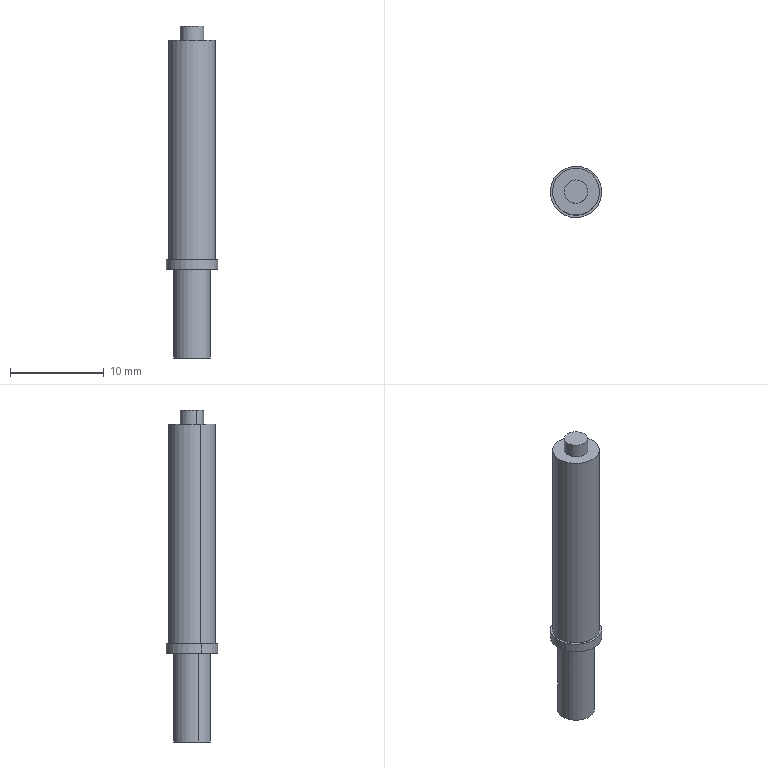Component | SolidWorks | 170423A4-ThimbleSpringGP-2T-1 | 1 solid | 17 faces | box 5.5 x 5.5 x 35.5 mm | volume 566 mm3 | cylinder 10 | plane 5 | cone 2 | commonest cylinder face diameters 2.5 x4 5 x2 5.5 x2 3.95 x2
build123d program:
from build123d import *

# Parameters (mm, degrees)
M3_TAPPED_HOLE1_D     = 2.5
M3_TAPPED_HOLE1_DEPTH = 8.5
M3_TAPPED_HOLE1_TIP   = 0.7511


with BuildPart() as part:
    # Sketch1 → Revolve1 (revolve)
    with BuildSketch(Plane(origin=(0, 0, 0), x_dir=(0, 0, -1), z_dir=(1, 0, 0))):
        Polygon((0, 35.5), (1.975, 35.5), (1.975, 26), (2.75, 26), (2.75, 25), (2.5, 25), (2.5, 1.5), (1.25, 1.5), (1.25, 0), (0, 0), align=None)
    revolve(axis=Axis((0, 0, 0), (0, 1, 0)))

    # M3 Tapped Hole1
    with Locations(Plane(origin=(0, 35.5, 0), x_dir=(-1, 0, 0), z_dir=(0, 1, 0))):
        with Locations((0, 0)):
            Hole(M3_TAPPED_HOLE1_D / 2, depth=M3_TAPPED_HOLE1_DEPTH)
            with Locations((0, 0, -(M3_TAPPED_HOLE1_DEPTH + M3_TAPPED_HOLE1_TIP / 2))):  # 118° drill point
                Cone(0, M3_TAPPED_HOLE1_D / 2, M3_TAPPED_HOLE1_TIP, mode=Mode.SUBTRACT)


solid = part.part

# Placed as in the assembly
solid = solid.moved(Location((66.187, 31.389, -54.574), (-90, 0, 0)))
STEP:
#1=COLOUR_RGB('',0.7922,0.8196,0.9333);
#2=FILL_AREA_STYLE_COLOUR('',#1);
#3=FILL_AREA_STYLE('',(#2));
#4=SURFACE_STYLE_FILL_AREA(#3);
#5=SURFACE_SIDE_STYLE('',(#4));
#6=SURFACE_STYLE_USAGE(.BOTH.,#5);
#7=PRESENTATION_STYLE_ASSIGNMENT((#6));
#8=CARTESIAN_POINT('',(2.651,1.254,-3.212));
#9=VERTEX_POINT('',#8);
#10=CARTESIAN_POINT('',(2.56,1.217,-3.212));
#11=VERTEX_POINT('',#10);
#12=CARTESIAN_POINT('',(2.606,1.236,-3.212));
#13=DIRECTION('',(-0.,0.,-1.));
#14=DIRECTION('',(-0.9265,-0.3763,0.));
#15=AXIS2_PLACEMENT_3D('',#12,#13,#14);
#16=CIRCLE('',#15,0.04921);
#17=EDGE_CURVE('',#9,#11,#16,.T.);
#18=ORIENTED_EDGE('',*,*,#17,.F.);
#19=CARTESIAN_POINT('',(2.651,1.254,-3.546));
#20=VERTEX_POINT('',#19);
#21=CARTESIAN_POINT('',(2.651,1.254,-3.546));
#22=DIRECTION('',(-0.,0.,-1.));
#23=VECTOR('',#22,39.37);
#24=LINE('',#21,#23);
#25=EDGE_CURVE('',#9,#20,#24,.T.);
#26=ORIENTED_EDGE('',*,*,#25,.T.);
#27=CARTESIAN_POINT('',(2.56,1.217,-3.546));
#28=VERTEX_POINT('',#27);
#29=CARTESIAN_POINT('',(2.606,1.236,-3.546));
#30=DIRECTION('',(-0.,0.,-1.));
#31=DIRECTION('',(-0.9265,-0.3763,0.));
#32=AXIS2_PLACEMENT_3D('',#29,#30,#31);
#33=CIRCLE('',#32,0.04921);
#34=EDGE_CURVE('',#20,#28,#33,.T.);
#35=ORIENTED_EDGE('',*,*,#34,.T.);
#36=CARTESIAN_POINT('',(2.56,1.217,-3.546));
#37=DIRECTION('',(-0.,0.,-1.));
#38=VECTOR('',#37,39.37);
#39=LINE('',#36,#38);
#40=EDGE_CURVE('',#11,#28,#39,.T.);
#41=ORIENTED_EDGE('',*,*,#40,.F.);
#42=EDGE_LOOP('',(#18,#26,#35,#41));
#43=FACE_OUTER_BOUND('',#42,.T.);
#44=CARTESIAN_POINT('',(2.606,1.236,-3.546));
#45=DIRECTION('',(-0.,0.,-1.));
#46=DIRECTION('',(-0.9265,-0.3763,0.));
#47=AXIS2_PLACEMENT_3D('',#44,#45,#46);
#48=CYLINDRICAL_SURFACE('',#47,0.04921);
#49=ADVANCED_FACE('',(#43),#48,.F.);
#50=CARTESIAN_POINT('',(2.606,1.236,-3.182));
#51=VERTEX_POINT('',#50);
#52=CARTESIAN_POINT('',(2.56,1.217,-3.212));
#53=DIRECTION('',(-0.7942,-0.3226,-0.515));
#54=VECTOR('',#53,39.37);
#55=LINE('',#52,#54);
#56=EDGE_CURVE('',#51,#11,#55,.T.);
#57=ORIENTED_EDGE('',*,*,#56,.F.);
#58=CARTESIAN_POINT('',(2.651,1.254,-3.212));
#59=DIRECTION('',(0.7942,0.3226,-0.515));
#60=VECTOR('',#59,39.37);
#61=LINE('',#58,#60);
#62=EDGE_CURVE('',#51,#9,#61,.T.);
#63=ORIENTED_EDGE('',*,*,#62,.T.);
#64=ORIENTED_EDGE('',*,*,#17,.T.);
#65=EDGE_LOOP('',(#57,#63,#64));
#66=FACE_OUTER_BOUND('',#65,.T.);
#67=CARTESIAN_POINT('',(2.606,1.236,-3.212));
#68=DIRECTION('',(-0.,0.,-1.));
#69=DIRECTION('',(-0.9265,-0.3763,0.));
#70=AXIS2_PLACEMENT_3D('',#67,#68,#69);
#71=CONICAL_SURFACE('',#70,0.04921,1.03);
#72=ADVANCED_FACE('',(#66),#71,.F.);
#73=CARTESIAN_POINT('',(2.651,1.254,-2.208));
#74=VERTEX_POINT('',#73);
#75=CARTESIAN_POINT('',(2.56,1.217,-2.208));
#76=VERTEX_POINT('',#75);
#77=CARTESIAN_POINT('',(2.606,1.236,-2.208));
#78=DIRECTION('',(0.,-0.,1.));
#79=DIRECTION('',(0.9265,0.3763,0.));
#80=AXIS2_PLACEMENT_3D('',#77,#78,#79);
#81=CIRCLE('',#80,0.04921);
#82=EDGE_CURVE('',#74,#76,#81,.T.);
#83=ORIENTED_EDGE('',*,*,#82,.T.);
#84=CARTESIAN_POINT('',(2.56,1.217,-2.149));
#85=VERTEX_POINT('',#84);
#86=CARTESIAN_POINT('',(2.56,1.217,-2.149));
#87=DIRECTION('',(0.,-0.,1.));
#88=VECTOR('',#87,39.37);
#89=LINE('',#86,#88);
#90=EDGE_CURVE('',#76,#85,#89,.T.);
#91=ORIENTED_EDGE('',*,*,#90,.T.);
#92=CARTESIAN_POINT('',(2.651,1.254,-2.149));
#93=VERTEX_POINT('',#92);
#94=CARTESIAN_POINT('',(2.606,1.236,-2.149));
#95=DIRECTION('',(0.,-0.,1.));
#96=DIRECTION('',(0.9265,0.3763,0.));
#97=AXIS2_PLACEMENT_3D('',#94,#95,#96);
#98=CIRCLE('',#97,0.04921);
#99=EDGE_CURVE('',#93,#85,#98,.T.);
#100=ORIENTED_EDGE('',*,*,#99,.F.);
#101=CARTESIAN_POINT('',(2.651,1.254,-2.149));
#102=DIRECTION('',(0.,-0.,1.));
#103=VECTOR('',#102,39.37);
#104=LINE('',#101,#103);
#105=EDGE_CURVE('',#74,#93,#104,.T.);
#106=ORIENTED_EDGE('',*,*,#105,.F.);
#107=EDGE_LOOP('',(#83,#91,#100,#106));
#108=FACE_OUTER_BOUND('',#107,.T.);
#109=CARTESIAN_POINT('',(2.606,1.236,-2.149));
#110=DIRECTION('',(0.,-0.,1.));
#111=DIRECTION('',(0.9265,0.3763,0.));
#112=AXIS2_PLACEMENT_3D('',#109,#110,#111);
#113=CYLINDRICAL_SURFACE('',#112,0.04921);
#114=ADVANCED_FACE('',(#108),#113,.T.);
#115=CARTESIAN_POINT('',(2.697,1.273,-3.133));
#116=VERTEX_POINT('',#115);
#117=CARTESIAN_POINT('',(2.515,1.199,-3.133));
#118=VERTEX_POINT('',#117);
#119=CARTESIAN_POINT('',(2.606,1.236,-3.133));
#120=DIRECTION('',(0.,-0.,1.));
#121=DIRECTION('',(0.9265,0.3763,0.));
#122=AXIS2_PLACEMENT_3D('',#119,#120,#121);
#123=CIRCLE('',#122,0.09843);
#124=EDGE_CURVE('',#116,#118,#123,.T.);
#125=ORIENTED_EDGE('',*,*,#124,.T.);
#126=CARTESIAN_POINT('',(2.515,1.199,-2.208));
#127=VERTEX_POINT('',#126);
#128=CARTESIAN_POINT('',(2.515,1.199,-2.149));
#129=DIRECTION('',(0.,-0.,1.));
#130=VECTOR('',#129,39.37);
#131=LINE('',#128,#130);
#132=EDGE_CURVE('',#118,#127,#131,.T.);
#133=ORIENTED_EDGE('',*,*,#132,.T.);
#134=CARTESIAN_POINT('',(2.697,1.273,-2.208));
#135=VERTEX_POINT('',#134);
#136=CARTESIAN_POINT('',(2.606,1.236,-2.208));
#137=DIRECTION('',(0.,-0.,1.));
#138=DIRECTION('',(0.9265,0.3763,0.));
#139=AXIS2_PLACEMENT_3D('',#136,#137,#138);
#140=CIRCLE('',#139,0.09843);
#141=EDGE_CURVE('',#135,#127,#140,.T.);
#142=ORIENTED_EDGE('',*,*,#141,.F.);
#143=CARTESIAN_POINT('',(2.697,1.273,-2.149));
#144=DIRECTION('',(0.,-0.,1.));
#145=VECTOR('',#144,39.37);
#146=LINE('',#143,#145);
#147=EDGE_CURVE('',#116,#135,#146,.T.);
#148=ORIENTED_EDGE('',*,*,#147,.F.);
#149=EDGE_LOOP('',(#125,#133,#142,#148));
#150=FACE_OUTER_BOUND('',#149,.T.);
#151=CARTESIAN_POINT('',(2.606,1.236,-2.149));
#152=DIRECTION('',(0.,-0.,1.));
#153=DIRECTION('',(0.9265,0.3763,0.));
#154=AXIS2_PLACEMENT_3D('',#151,#152,#153);
#155=CYLINDRICAL_SURFACE('',#154,0.09843);
#156=ADVANCED_FACE('',(#150),#155,.T.);
#157=CARTESIAN_POINT('',(2.706,1.277,-3.172));
#158=VERTEX_POINT('',#157);
#159=CARTESIAN_POINT('',(2.505,1.195,-3.172));
#160=VERTEX_POINT('',#159);
#161=CARTESIAN_POINT('',(2.606,1.236,-3.172));
#162=DIRECTION('',(0.,-0.,1.));
#163=DIRECTION('',(0.9265,0.3763,0.));
#164=AXIS2_PLACEMENT_3D('',#161,#162,#163);
#165=CIRCLE('',#164,0.1083);
#166=EDGE_CURVE('',#158,#160,#165,.T.);
#167=ORIENTED_EDGE('',*,*,#166,.T.);
#168=CARTESIAN_POINT('',(2.505,1.195,-3.133));
#169=VERTEX_POINT('',#168);
#170=CARTESIAN_POINT('',(2.505,1.195,-2.149));
#171=DIRECTION('',(0.,-0.,1.));
#172=VECTOR('',#171,39.37);
#173=LINE('',#170,#172);
#174=EDGE_CURVE('',#160,#169,#173,.T.);
#175=ORIENTED_EDGE('',*,*,#174,.T.);
#176=CARTESIAN_POINT('',(2.706,1.277,-3.133));
#177=VERTEX_POINT('',#176);
#178=CARTESIAN_POINT('',(2.606,1.236,-3.133));
#179=DIRECTION('',(0.,-0.,1.));
#180=DIRECTION('',(0.9265,0.3763,0.));
#181=AXIS2_PLACEMENT_3D('',#178,#179,#180);
#182=CIRCLE('',#181,0.1083);
#183=EDGE_CURVE('',#177,#169,#182,.T.);
#184=ORIENTED_EDGE('',*,*,#183,.F.);
#185=CARTESIAN_POINT('',(2.706,1.277,-2.149));
#186=DIRECTION('',(0.,-0.,1.));
#187=VECTOR('',#186,39.37);
#188=LINE('',#185,#187);
#189=EDGE_CURVE('',#158,#177,#188,.T.);
#190=ORIENTED_EDGE('',*,*,#189,.F.);
#191=EDGE_LOOP('',(#167,#175,#184,#190));
#192=FACE_OUTER_BOUND('',#191,.T.);
#193=CARTESIAN_POINT('',(2.606,1.236,-2.149));
#194=DIRECTION('',(0.,-0.,1.));
#195=DIRECTION('',(0.9265,0.3763,0.));
#196=AXIS2_PLACEMENT_3D('',#193,#194,#195);
#197=CYLINDRICAL_SURFACE('',#196,0.1083);
#198=ADVANCED_FACE('',(#192),#197,.T.);
#199=CARTESIAN_POINT('',(2.678,1.265,-3.546));
#200=VERTEX_POINT('',#199);
#201=CARTESIAN_POINT('',(2.534,1.207,-3.546));
#202=VERTEX_POINT('',#201);
#203=CARTESIAN_POINT('',(2.606,1.236,-3.546));
#204=DIRECTION('',(0.,-0.,1.));
#205=DIRECTION('',(0.9265,0.3763,0.));
#206=AXIS2_PLACEMENT_3D('',#203,#204,#205);
#207=CIRCLE('',#206,0.07776);
#208=EDGE_CURVE('',#200,#202,#207,.T.);
#209=ORIENTED_EDGE('',*,*,#208,.T.);
#210=CARTESIAN_POINT('',(2.534,1.207,-3.172));
#211=VERTEX_POINT('',#210);
#212=CARTESIAN_POINT('',(2.534,1.207,-2.149));
#213=DIRECTION('',(0.,-0.,1.));
#214=VECTOR('',#213,39.37);
#215=LINE('',#212,#214);
#216=EDGE_CURVE('',#202,#211,#215,.T.);
#217=ORIENTED_EDGE('',*,*,#216,.T.);
#218=CARTESIAN_POINT('',(2.678,1.265,-3.172));
#219=VERTEX_POINT('',#218);
#220=CARTESIAN_POINT('',(2.606,1.236,-3.172));
#221=DIRECTION('',(0.,-0.,1.));
#222=DIRECTION('',(0.9265,0.3763,0.));
#223=AXIS2_PLACEMENT_3D('',#220,#221,#222);
#224=CIRCLE('',#223,0.07776);
#225=EDGE_CURVE('',#219,#211,#224,.T.);
#226=ORIENTED_EDGE('',*,*,#225,.F.);
#227=CARTESIAN_POINT('',(2.678,1.265,-2.149));
#228=DIRECTION('',(0.,-0.,1.));
#229=VECTOR('',#228,39.37);
#230=LINE('',#227,#229);
#231=EDGE_CURVE('',#200,#219,#230,.T.);
#232=ORIENTED_EDGE('',*,*,#231,.F.);
#233=EDGE_LOOP('',(#209,#217,#226,#232));
#234=FACE_OUTER_BOUND('',#233,.T.);
#235=CARTESIAN_POINT('',(2.606,1.236,-2.149));
#236=DIRECTION('',(0.,-0.,1.));
#237=DIRECTION('',(0.9265,0.3763,0.));
#238=AXIS2_PLACEMENT_3D('',#235,#236,#237);
#239=CYLINDRICAL_SURFACE('',#238,0.07776);
#240=ADVANCED_FACE('',(#234),#239,.T.);
#241=CARTESIAN_POINT('',(2.606,1.236,-3.546));
#242=DIRECTION('',(-0.,0.,-1.));
#243=DIRECTION('',(-0.9265,-0.3763,0.));
#244=AXIS2_PLACEMENT_3D('',#241,#242,#243);
#245=CIRCLE('',#244,0.04921);
#246=EDGE_CURVE('',#28,#20,#245,.T.);
#247=ORIENTED_EDGE('',*,*,#246,.F.);
#248=ORIENTED_EDGE('',*,*,#34,.F.);
#249=EDGE_LOOP('',(#247,#248));
#250=FACE_BOUND('',#249,.T.);
#251=ORIENTED_EDGE('',*,*,#208,.F.);
#252=CARTESIAN_POINT('',(2.606,1.236,-3.546));
#253=DIRECTION('',(0.,-0.,1.));
#254=DIRECTION('',(0.9265,0.3763,0.));
#255=AXIS2_PLACEMENT_3D('',#252,#253,#254);
#256=CIRCLE('',#255,0.07776);
#257=EDGE_CURVE('',#202,#200,#256,.T.);
#258=ORIENTED_EDGE('',*,*,#257,.F.);
#259=EDGE_LOOP('',(#251,#258));
#260=FACE_OUTER_BOUND('',#259,.T.);
#261=CARTESIAN_POINT('',(2.606,1.236,-3.546));
#262=DIRECTION('',(-0.,0.,-1.));
#263=DIRECTION('',(-0.9265,-0.3763,-0.));
#264=AXIS2_PLACEMENT_3D('',#261,#262,#263);
#265=PLANE('',#264);
#266=ADVANCED_FACE('',(#250,#260),#265,.T.);
#267=ORIENTED_EDGE('',*,*,#216,.F.);
#268=ORIENTED_EDGE('',*,*,#257,.T.);
#269=ORIENTED_EDGE('',*,*,#231,.T.);
#270=CARTESIAN_POINT('',(2.606,1.236,-3.172));
#271=DIRECTION('',(0.,-0.,1.));
#272=DIRECTION('',(0.9265,0.3763,0.));
#273=AXIS2_PLACEMENT_3D('',#270,#271,#272);
#274=CIRCLE('',#273,0.07776);
#275=EDGE_CURVE('',#211,#219,#274,.T.);
#276=ORIENTED_EDGE('',*,*,#275,.F.);
#277=EDGE_LOOP('',(#267,#268,#269,#276));
#278=FACE_OUTER_BOUND('',#277,.T.);
#279=CARTESIAN_POINT('',(2.606,1.236,-2.149));
#280=DIRECTION('',(0.,-0.,1.));
#281=DIRECTION('',(0.9265,0.3763,0.));
#282=AXIS2_PLACEMENT_3D('',#279,#280,#281);
#283=CYLINDRICAL_SURFACE('',#282,0.07776);
#284=ADVANCED_FACE('',(#278),#283,.T.);
#285=ORIENTED_EDGE('',*,*,#225,.T.);
#286=ORIENTED_EDGE('',*,*,#275,.T.);
#287=EDGE_LOOP('',(#285,#286));
#288=FACE_BOUND('',#287,.T.);
#289=ORIENTED_EDGE('',*,*,#166,.F.);
#290=CARTESIAN_POINT('',(2.606,1.236,-3.172));
#291=DIRECTION('',(0.,-0.,1.));
#292=DIRECTION('',(0.9265,0.3763,0.));
#293=AXIS2_PLACEMENT_3D('',#290,#291,#292);
#294=CIRCLE('',#293,0.1083);
#295=EDGE_CURVE('',#160,#158,#294,.T.);
#296=ORIENTED_EDGE('',*,*,#295,.F.);
#297=EDGE_LOOP('',(#289,#296));
#298=FACE_OUTER_BOUND('',#297,.T.);
#299=CARTESIAN_POINT('',(2.678,1.265,-3.172));
#300=DIRECTION('',(-0.,0.,-1.));
#301=DIRECTION('',(-0.9265,-0.3763,-0.));
#302=AXIS2_PLACEMENT_3D('',#299,#300,#301);
#303=PLANE('',#302);
#304=ADVANCED_FACE('',(#288,#298),#303,.T.);
#305=ORIENTED_EDGE('',*,*,#174,.F.);
#306=ORIENTED_EDGE('',*,*,#295,.T.);
#307=ORIENTED_EDGE('',*,*,#189,.T.);
#308=CARTESIAN_POINT('',(2.606,1.236,-3.133));
#309=DIRECTION('',(0.,-0.,1.));
#310=DIRECTION('',(0.9265,0.3763,0.));
#311=AXIS2_PLACEMENT_3D('',#308,#309,#310);
#312=CIRCLE('',#311,0.1083);
#313=EDGE_CURVE('',#169,#177,#312,.T.);
#314=ORIENTED_EDGE('',*,*,#313,.F.);
#315=EDGE_LOOP('',(#305,#306,#307,#314));
#316=FACE_OUTER_BOUND('',#315,.T.);
#317=CARTESIAN_POINT('',(2.606,1.236,-2.149));
#318=DIRECTION('',(0.,-0.,1.));
#319=DIRECTION('',(0.9265,0.3763,0.));
#320=AXIS2_PLACEMENT_3D('',#317,#318,#319);
#321=CYLINDRICAL_SURFACE('',#320,0.1083);
#322=ADVANCED_FACE('',(#316),#321,.T.);
#323=ORIENTED_EDGE('',*,*,#183,.T.);
#324=ORIENTED_EDGE('',*,*,#313,.T.);
#325=EDGE_LOOP('',(#323,#324));
#326=FACE_OUTER_BOUND('',#325,.T.);
#327=ORIENTED_EDGE('',*,*,#124,.F.);
#328=CARTESIAN_POINT('',(2.606,1.236,-3.133));
#329=DIRECTION('',(0.,-0.,1.));
#330=DIRECTION('',(0.9265,0.3763,0.));
#331=AXIS2_PLACEMENT_3D('',#328,#329,#330);
#332=CIRCLE('',#331,0.09843);
#333=EDGE_CURVE('',#118,#116,#332,.T.);
#334=ORIENTED_EDGE('',*,*,#333,.F.);
#335=EDGE_LOOP('',(#327,#334));
#336=FACE_BOUND('',#335,.T.);
#337=CARTESIAN_POINT('',(2.706,1.277,-3.133));
#338=DIRECTION('',(0.,-0.,1.));
#339=DIRECTION('',(0.9265,0.3763,0.));
#340=AXIS2_PLACEMENT_3D('',#337,#338,#339);
#341=PLANE('',#340);
#342=ADVANCED_FACE('',(#326,#336),#341,.T.);
#343=ORIENTED_EDGE('',*,*,#132,.F.);
#344=ORIENTED_EDGE('',*,*,#333,.T.);
#345=ORIENTED_EDGE('',*,*,#147,.T.);
#346=CARTESIAN_POINT('',(2.606,1.236,-2.208));
#347=DIRECTION('',(0.,-0.,1.));
#348=DIRECTION('',(0.9265,0.3763,0.));
#349=AXIS2_PLACEMENT_3D('',#346,#347,#348);
#350=CIRCLE('',#349,0.09843);
#351=EDGE_CURVE('',#127,#135,#350,.T.);
#352=ORIENTED_EDGE('',*,*,#351,.F.);
#353=EDGE_LOOP('',(#343,#344,#345,#352));
#354=FACE_OUTER_BOUND('',#353,.T.);
#355=CARTESIAN_POINT('',(2.606,1.236,-2.149));
#356=DIRECTION('',(0.,-0.,1.));
#357=DIRECTION('',(0.9265,0.3763,0.));
#358=AXIS2_PLACEMENT_3D('',#355,#356,#357);
#359=CYLINDRICAL_SURFACE('',#358,0.09843);
#360=ADVANCED_FACE('',(#354),#359,.T.);
#361=ORIENTED_EDGE('',*,*,#141,.T.);
#362=ORIENTED_EDGE('',*,*,#351,.T.);
#363=EDGE_LOOP('',(#361,#362));
#364=FACE_OUTER_BOUND('',#363,.T.);
#365=ORIENTED_EDGE('',*,*,#82,.F.);
#366=CARTESIAN_POINT('',(2.606,1.236,-2.208));
#367=DIRECTION('',(0.,-0.,1.));
#368=DIRECTION('',(0.9265,0.3763,0.));
#369=AXIS2_PLACEMENT_3D('',#366,#367,#368);
#370=CIRCLE('',#369,0.04921);
#371=EDGE_CURVE('',#76,#74,#370,.T.);
#372=ORIENTED_EDGE('',*,*,#371,.F.);
#373=EDGE_LOOP('',(#365,#372));
#374=FACE_BOUND('',#373,.T.);
#375=CARTESIAN_POINT('',(2.697,1.273,-2.208));
#376=DIRECTION('',(0.,-0.,1.));
#377=DIRECTION('',(0.9265,0.3763,0.));
#378=AXIS2_PLACEMENT_3D('',#375,#376,#377);
#379=PLANE('',#378);
#380=ADVANCED_FACE('',(#364,#374),#379,.T.);
#381=ORIENTED_EDGE('',*,*,#90,.F.);
#382=ORIENTED_EDGE('',*,*,#371,.T.);
#383=ORIENTED_EDGE('',*,*,#105,.T.);
#384=CARTESIAN_POINT('',(2.606,1.236,-2.149));
#385=DIRECTION('',(0.,-0.,1.));
#386=DIRECTION('',(0.9265,0.3763,0.));
#387=AXIS2_PLACEMENT_3D('',#384,#385,#386);
#388=CIRCLE('',#387,0.04921);
#389=EDGE_CURVE('',#85,#93,#388,.T.);
#390=ORIENTED_EDGE('',*,*,#389,.F.);
#391=EDGE_LOOP('',(#381,#382,#383,#390));
#392=FACE_OUTER_BOUND('',#391,.T.);
#393=CARTESIAN_POINT('',(2.606,1.236,-2.149));
#394=DIRECTION('',(0.,-0.,1.));
#395=DIRECTION('',(0.9265,0.3763,0.));
#396=AXIS2_PLACEMENT_3D('',#393,#394,#395);
#397=CYLINDRICAL_SURFACE('',#396,0.04921);
#398=ADVANCED_FACE('',(#392),#397,.T.);
#399=ORIENTED_EDGE('',*,*,#99,.T.);
#400=ORIENTED_EDGE('',*,*,#389,.T.);
#401=EDGE_LOOP('',(#399,#400));
#402=FACE_OUTER_BOUND('',#401,.T.);
#403=CARTESIAN_POINT('',(2.651,1.254,-2.149));
#404=DIRECTION('',(0.,-0.,1.));
#405=DIRECTION('',(0.9265,0.3763,0.));
#406=AXIS2_PLACEMENT_3D('',#403,#404,#405);
#407=PLANE('',#406);
#408=ADVANCED_FACE('',(#402),#407,.T.);
#409=ORIENTED_EDGE('',*,*,#62,.F.);
#410=ORIENTED_EDGE('',*,*,#56,.T.);
#411=CARTESIAN_POINT('',(2.606,1.236,-3.212));
#412=DIRECTION('',(-0.,0.,-1.));
#413=DIRECTION('',(-0.9265,-0.3763,0.));
#414=AXIS2_PLACEMENT_3D('',#411,#412,#413);
#415=CIRCLE('',#414,0.04921);
#416=EDGE_CURVE('',#11,#9,#415,.T.);
#417=ORIENTED_EDGE('',*,*,#416,.T.);
#418=EDGE_LOOP('',(#409,#410,#417));
#419=FACE_OUTER_BOUND('',#418,.T.);
#420=CARTESIAN_POINT('',(2.606,1.236,-3.212));
#421=DIRECTION('',(-0.,0.,-1.));
#422=DIRECTION('',(-0.9265,-0.3763,0.));
#423=AXIS2_PLACEMENT_3D('',#420,#421,#422);
#424=CONICAL_SURFACE('',#423,0.04921,1.03);
#425=ADVANCED_FACE('',(#419),#424,.F.);
#426=ORIENTED_EDGE('',*,*,#25,.F.);
#427=ORIENTED_EDGE('',*,*,#416,.F.);
#428=ORIENTED_EDGE('',*,*,#40,.T.);
#429=ORIENTED_EDGE('',*,*,#246,.T.);
#430=EDGE_LOOP('',(#426,#427,#428,#429));
#431=FACE_OUTER_BOUND('',#430,.T.);
#432=CARTESIAN_POINT('',(2.606,1.236,-3.546));
#433=DIRECTION('',(-0.,0.,-1.));
#434=DIRECTION('',(-0.9265,-0.3763,0.));
#435=AXIS2_PLACEMENT_3D('',#432,#433,#434);
#436=CYLINDRICAL_SURFACE('',#435,0.04921);
#437=ADVANCED_FACE('',(#431),#436,.F.);
#438=CLOSED_SHELL('',(#49,#72,#114,#156,#198,#240,#266,#284,#304,#322,#342,#360,#380,#398,#408,#425,#437));
#439=MANIFOLD_SOLID_BREP('',#438);
#440=STYLED_ITEM('',(#7),#439);
#441=PRESENTATION_LAYER_ASSIGNMENT('','',(#440));
#442=CARTESIAN_POINT('',(0.,0.,0.));
#443=DIRECTION('',(0.,0.,1.));
#444=DIRECTION('',(1.,0.,0.));
#445=AXIS2_PLACEMENT_3D('',#442,#443,#444);
#446=(LENGTH_UNIT()NAMED_UNIT(*)SI_UNIT($,.METRE.));
#447=LENGTH_MEASURE_WITH_UNIT(LENGTH_MEASURE(0.0254),#446);
#448=DIMENSIONAL_EXPONENTS(1.,0.,0.,0.,0.,0.,0.);
#449=(CONVERSION_BASED_UNIT('',#447)LENGTH_UNIT()NAMED_UNIT(#448));
#450=UNCERTAINTY_MEASURE_WITH_UNIT(LENGTH_MEASURE(0.00001),#449,'','');
#451=(NAMED_UNIT(*)PLANE_ANGLE_UNIT()SI_UNIT($,.RADIAN.));
#452=(NAMED_UNIT(*)SI_UNIT($,.STERADIAN.)SOLID_ANGLE_UNIT());
#453=(GEOMETRIC_REPRESENTATION_CONTEXT(3)GLOBAL_UNCERTAINTY_ASSIGNED_CONTEXT((#450))GLOBAL_UNIT_ASSIGNED_CONTEXT((#449,#451,#452))REPRESENTATION_CONTEXT('',''));
#454=ADVANCED_BREP_SHAPE_REPRESENTATION('',(#439,#445),#453);
#455=(LENGTH_UNIT()NAMED_UNIT(*)SI_UNIT($,.METRE.));
#456=LENGTH_MEASURE_WITH_UNIT(LENGTH_MEASURE(0.0254),#455);
#457=DIMENSIONAL_EXPONENTS(1.,0.,0.,0.,0.,0.,0.);
#458=(CONVERSION_BASED_UNIT('',#456)LENGTH_UNIT()NAMED_UNIT(#457));
#459=UNCERTAINTY_MEASURE_WITH_UNIT(LENGTH_MEASURE(0.00001),#458,'','');
#460=(NAMED_UNIT(*)PLANE_ANGLE_UNIT()SI_UNIT($,.RADIAN.));
#461=(NAMED_UNIT(*)SI_UNIT($,.STERADIAN.)SOLID_ANGLE_UNIT());
#462=(GEOMETRIC_REPRESENTATION_CONTEXT(3)GLOBAL_UNCERTAINTY_ASSIGNED_CONTEXT((#459))GLOBAL_UNIT_ASSIGNED_CONTEXT((#458,#460,#461))REPRESENTATION_CONTEXT('',''));
#463=MECHANICAL_DESIGN_GEOMETRIC_PRESENTATION_REPRESENTATION('',(#440),#462);